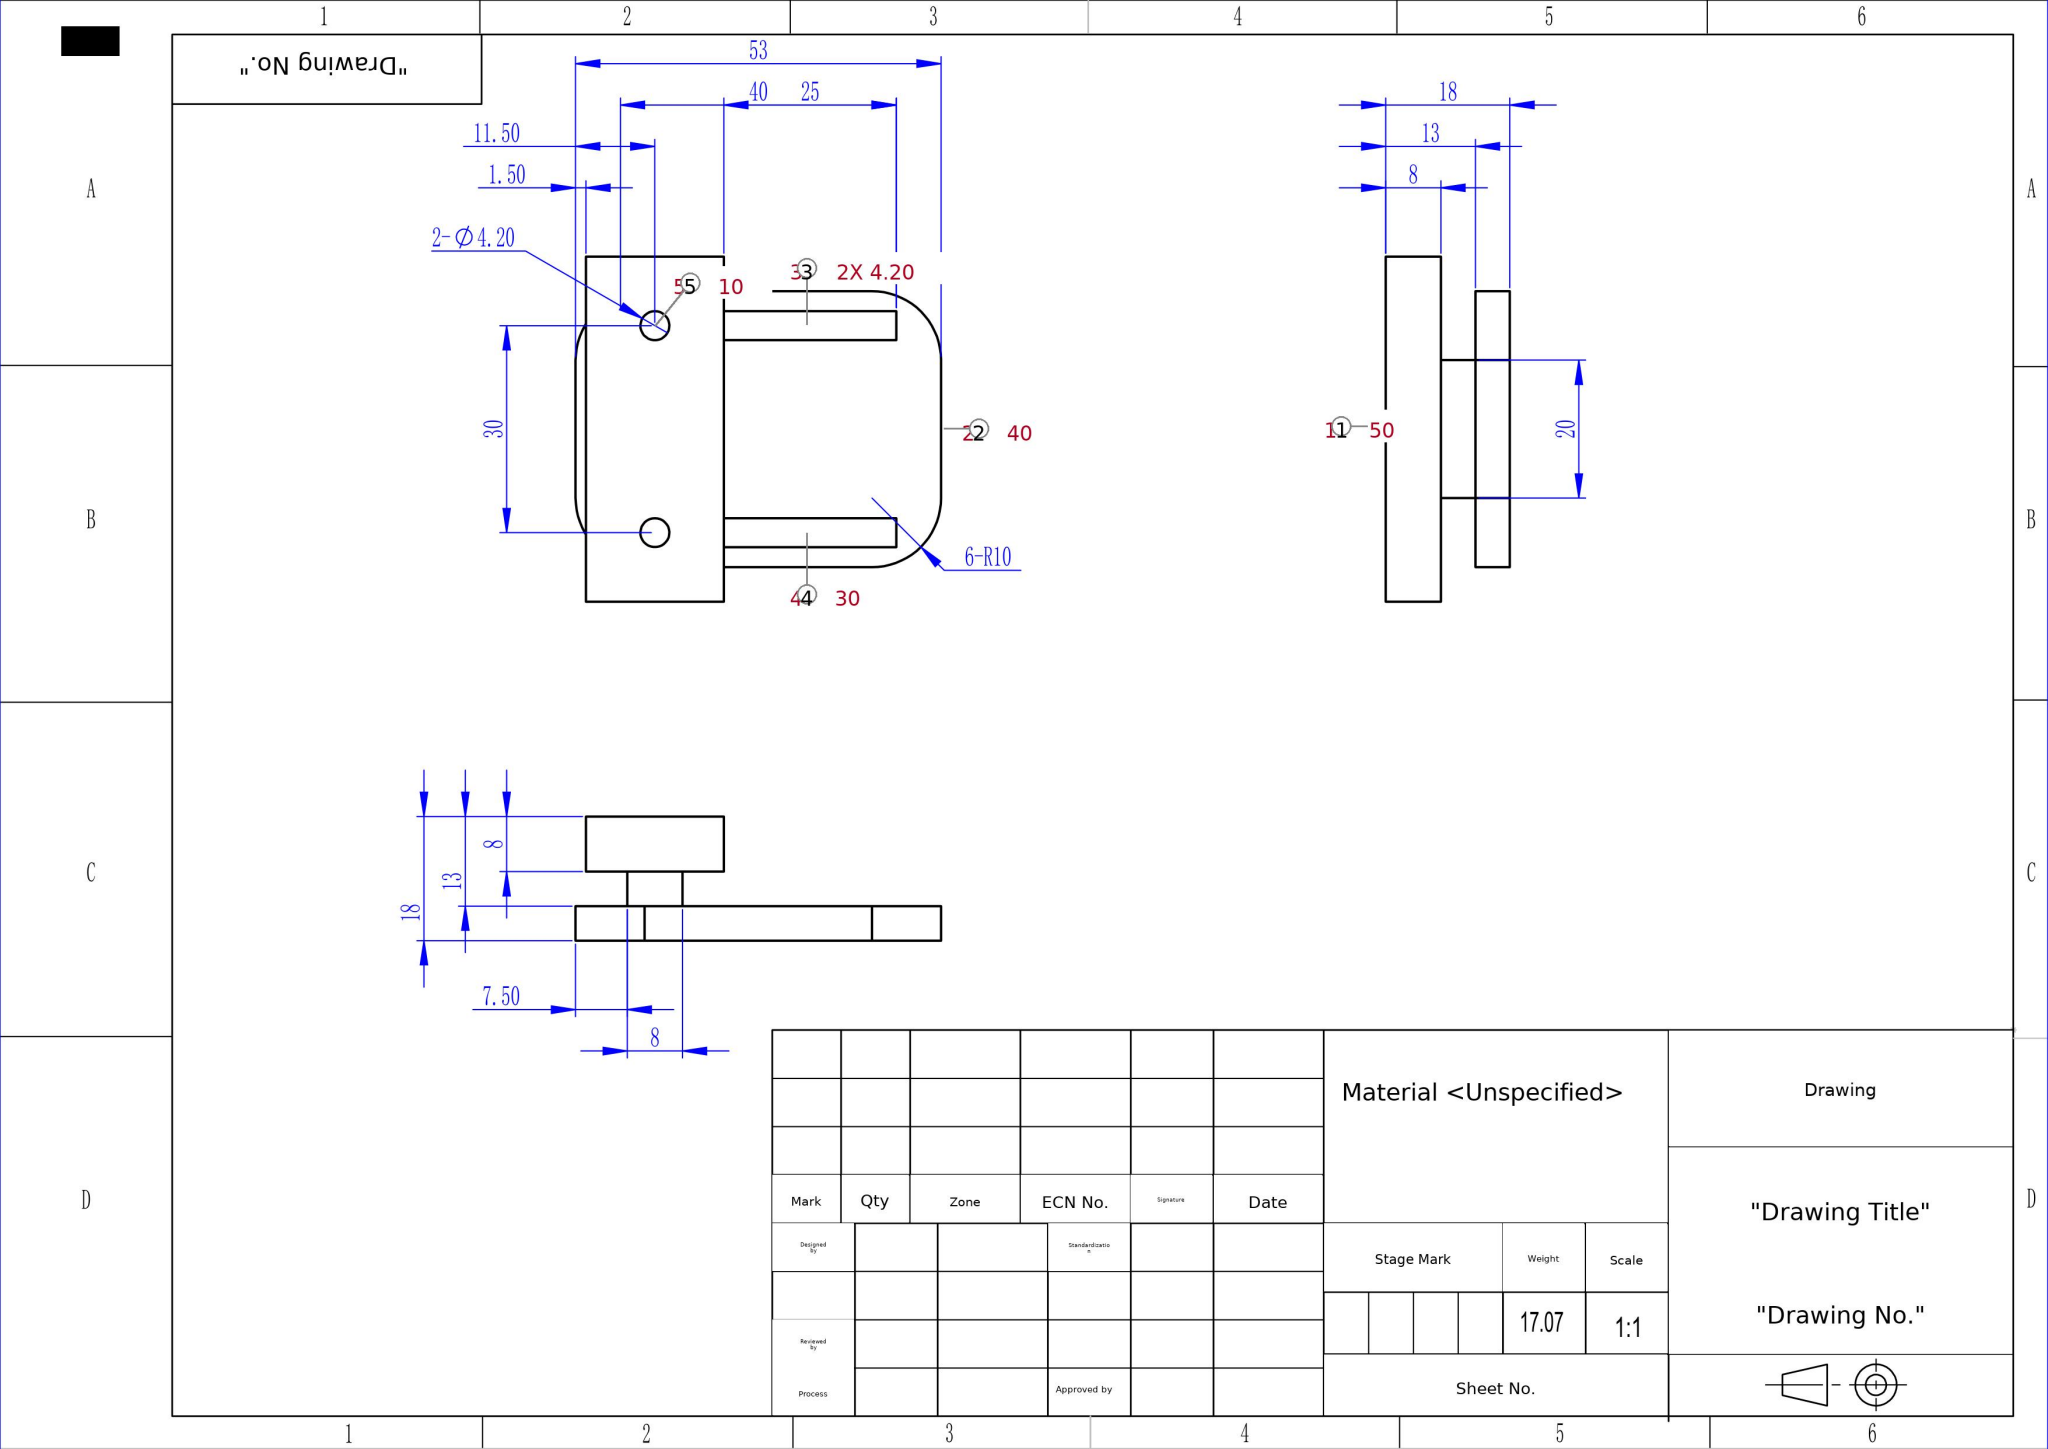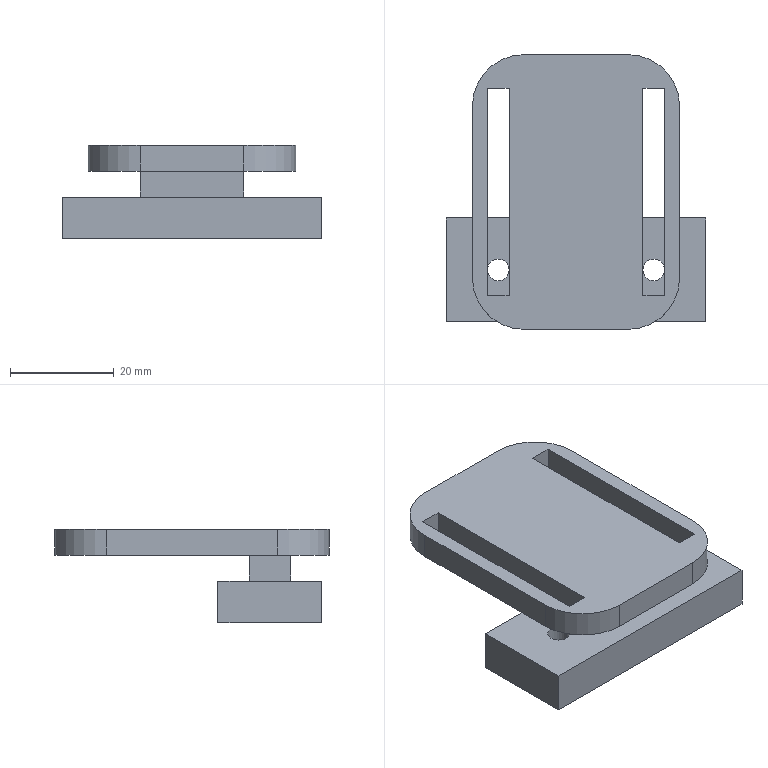Part | SolidWorks | mm | material Unspecified | 1 solid | 32 faces | box 50 x 53 x 18 mm | volume 17069 mm3 | plane 24 | cylinder 8 | commonest cylinder face diameters 4.2 x4 20 x4
build123d program:
from build123d import *

# Parameters (mm, degrees)
SKETCH1_W           = 50
SKETCH1_H           = 20
SKETCH1_R           = 2.1
BOSS_EXTRUDE1_DEPTH = 8
SKETCH2_W           = 20
SKETCH2_H           = 8
BOSS_EXTRUDE2_DEPTH = 5
SKETCH3_W           = 40
SKETCH3_H           = 53
SKETCH3_W_2         = 4.2
SKETCH3_H_2         = 40
BOSS_EXTRUDE3_DEPTH = 5
FILLET1_R           = 10


with BuildPart() as part:
    # Sketch1 → Boss-Extrude1 (new body)
    with BuildSketch(Plane.XY):
        Rectangle(SKETCH1_W, SKETCH1_H)
        with Locations((-15, 0)):
            Circle(SKETCH1_R, mode=Mode.SUBTRACT)
        with Locations((15, 0)):
            Circle(SKETCH1_R, mode=Mode.SUBTRACT)
    extrude(amount=BOSS_EXTRUDE1_DEPTH)

    # Sketch2 → Boss-Extrude2 (add)
    with BuildSketch(Plane.XY.offset(8)):
        Rectangle(SKETCH2_W, SKETCH2_H)
    extrude(amount=BOSS_EXTRUDE2_DEPTH)

    # Sketch3 → Boss-Extrude3 (add)
    with BuildSketch(Plane.XY.offset(13)):
        with Locations((0, 15)):
            Rectangle(SKETCH3_W, SKETCH3_H)
        with Locations((-15, 15)):
            Rectangle(SKETCH3_W_2, SKETCH3_H_2, mode=Mode.SUBTRACT)
        with Locations((15, 15)):
            Rectangle(SKETCH3_W_2, SKETCH3_H_2, mode=Mode.SUBTRACT)
    extrude(amount=BOSS_EXTRUDE3_DEPTH)

    # Fillet1
    fillet1_edges = [part.edges().sort_by_distance(p)[0] for p in [
        (20, -11.5, 15.5),
        (20, 41.5, 15.5),
        (-20, 41.5, 15.5),
        (-20, -11.5, 15.5),
    ]]
    fillet(fillet1_edges, radius=FILLET1_R)


solid = part.part
STEP:
#1=CARTESIAN_POINT('',(12.9,0.,8.));
#2=VERTEX_POINT('',#1);
#3=CARTESIAN_POINT('',(17.1,0.,8.));
#4=VERTEX_POINT('',#3);
#5=CARTESIAN_POINT('',(15.,0.,8.));
#6=DIRECTION('',(0.,0.,1.));
#7=DIRECTION('',(1.,0.,0.));
#8=AXIS2_PLACEMENT_3D('',#5,#6,#7);
#9=CIRCLE('',#8,2.1);
#10=EDGE_CURVE('',#2,#4,#9,.T.);
#11=ORIENTED_EDGE('',*,*,#10,.T.);
#12=CARTESIAN_POINT('',(17.1,0.,0.));
#13=VERTEX_POINT('',#12);
#14=CARTESIAN_POINT('',(17.1,0.,8.));
#15=DIRECTION('',(0.,0.,-1.));
#16=VECTOR('',#15,1000.);
#17=LINE('',#14,#16);
#18=EDGE_CURVE('',#4,#13,#17,.T.);
#19=ORIENTED_EDGE('',*,*,#18,.T.);
#20=CARTESIAN_POINT('',(12.9,0.,0.));
#21=VERTEX_POINT('',#20);
#22=CARTESIAN_POINT('',(15.,0.,0.));
#23=DIRECTION('',(0.,0.,1.));
#24=DIRECTION('',(1.,0.,0.));
#25=AXIS2_PLACEMENT_3D('',#22,#23,#24);
#26=CIRCLE('',#25,2.1);
#27=EDGE_CURVE('',#21,#13,#26,.T.);
#28=ORIENTED_EDGE('',*,*,#27,.F.);
#29=CARTESIAN_POINT('',(12.9,0.,8.));
#30=DIRECTION('',(0.,0.,-1.));
#31=VECTOR('',#30,1000.);
#32=LINE('',#29,#31);
#33=EDGE_CURVE('',#2,#21,#32,.T.);
#34=ORIENTED_EDGE('',*,*,#33,.F.);
#35=EDGE_LOOP('',(#11,#19,#28,#34));
#36=FACE_OUTER_BOUND('',#35,.T.);
#37=CARTESIAN_POINT('',(15.,0.,8.));
#38=DIRECTION('',(0.,0.,-1.));
#39=DIRECTION('',(-1.,0.,0.));
#40=AXIS2_PLACEMENT_3D('',#37,#38,#39);
#41=CYLINDRICAL_SURFACE('',#40,2.1);
#42=ADVANCED_FACE('',(#36),#41,.F.);
#43=CARTESIAN_POINT('',(-17.1,0.,8.));
#44=VERTEX_POINT('',#43);
#45=CARTESIAN_POINT('',(-12.9,0.,8.));
#46=VERTEX_POINT('',#45);
#47=CARTESIAN_POINT('',(-15.,0.,8.));
#48=DIRECTION('',(0.,0.,1.));
#49=DIRECTION('',(1.,0.,0.));
#50=AXIS2_PLACEMENT_3D('',#47,#48,#49);
#51=CIRCLE('',#50,2.1);
#52=EDGE_CURVE('',#44,#46,#51,.T.);
#53=ORIENTED_EDGE('',*,*,#52,.T.);
#54=CARTESIAN_POINT('',(-12.9,0.,0.));
#55=VERTEX_POINT('',#54);
#56=CARTESIAN_POINT('',(-12.9,0.,8.));
#57=DIRECTION('',(0.,0.,-1.));
#58=VECTOR('',#57,1000.);
#59=LINE('',#56,#58);
#60=EDGE_CURVE('',#46,#55,#59,.T.);
#61=ORIENTED_EDGE('',*,*,#60,.T.);
#62=CARTESIAN_POINT('',(-17.1,0.,0.));
#63=VERTEX_POINT('',#62);
#64=CARTESIAN_POINT('',(-15.,0.,0.));
#65=DIRECTION('',(0.,0.,1.));
#66=DIRECTION('',(1.,0.,0.));
#67=AXIS2_PLACEMENT_3D('',#64,#65,#66);
#68=CIRCLE('',#67,2.1);
#69=EDGE_CURVE('',#63,#55,#68,.T.);
#70=ORIENTED_EDGE('',*,*,#69,.F.);
#71=CARTESIAN_POINT('',(-17.1,0.,8.));
#72=DIRECTION('',(0.,0.,-1.));
#73=VECTOR('',#72,1000.);
#74=LINE('',#71,#73);
#75=EDGE_CURVE('',#44,#63,#74,.T.);
#76=ORIENTED_EDGE('',*,*,#75,.F.);
#77=EDGE_LOOP('',(#53,#61,#70,#76));
#78=FACE_OUTER_BOUND('',#77,.T.);
#79=CARTESIAN_POINT('',(-15.,0.,8.));
#80=DIRECTION('',(0.,0.,-1.));
#81=DIRECTION('',(-1.,0.,0.));
#82=AXIS2_PLACEMENT_3D('',#79,#80,#81);
#83=CYLINDRICAL_SURFACE('',#82,2.1);
#84=ADVANCED_FACE('',(#78),#83,.F.);
#85=ORIENTED_EDGE('',*,*,#52,.F.);
#86=CARTESIAN_POINT('',(-15.,0.,8.));
#87=DIRECTION('',(0.,0.,1.));
#88=DIRECTION('',(1.,0.,0.));
#89=AXIS2_PLACEMENT_3D('',#86,#87,#88);
#90=CIRCLE('',#89,2.1);
#91=EDGE_CURVE('',#46,#44,#90,.T.);
#92=ORIENTED_EDGE('',*,*,#91,.F.);
#93=EDGE_LOOP('',(#85,#92));
#94=FACE_BOUND('',#93,.T.);
#95=CARTESIAN_POINT('',(25.,-10.,8.));
#96=VERTEX_POINT('',#95);
#97=CARTESIAN_POINT('',(25.,10.,8.));
#98=VERTEX_POINT('',#97);
#99=CARTESIAN_POINT('',(25.,10.,8.));
#100=DIRECTION('',(-0.,1.,0.));
#101=VECTOR('',#100,1000.);
#102=LINE('',#99,#101);
#103=EDGE_CURVE('',#96,#98,#102,.T.);
#104=ORIENTED_EDGE('',*,*,#103,.T.);
#105=CARTESIAN_POINT('',(-25.,10.,8.));
#106=VERTEX_POINT('',#105);
#107=CARTESIAN_POINT('',(-25.,10.,8.));
#108=DIRECTION('',(-1.,0.,0.));
#109=VECTOR('',#108,1000.);
#110=LINE('',#107,#109);
#111=EDGE_CURVE('',#98,#106,#110,.T.);
#112=ORIENTED_EDGE('',*,*,#111,.T.);
#113=CARTESIAN_POINT('',(-25.,-10.,8.));
#114=VERTEX_POINT('',#113);
#115=CARTESIAN_POINT('',(-25.,10.,8.));
#116=DIRECTION('',(0.,-1.,0.));
#117=VECTOR('',#116,1000.);
#118=LINE('',#115,#117);
#119=EDGE_CURVE('',#106,#114,#118,.T.);
#120=ORIENTED_EDGE('',*,*,#119,.T.);
#121=CARTESIAN_POINT('',(-25.,-10.,8.));
#122=DIRECTION('',(1.,0.,0.));
#123=VECTOR('',#122,1000.);
#124=LINE('',#121,#123);
#125=EDGE_CURVE('',#114,#96,#124,.T.);
#126=ORIENTED_EDGE('',*,*,#125,.T.);
#127=EDGE_LOOP('',(#104,#112,#120,#126));
#128=FACE_OUTER_BOUND('',#127,.T.);
#129=ORIENTED_EDGE('',*,*,#10,.F.);
#130=CARTESIAN_POINT('',(15.,0.,8.));
#131=DIRECTION('',(0.,0.,1.));
#132=DIRECTION('',(1.,0.,0.));
#133=AXIS2_PLACEMENT_3D('',#130,#131,#132);
#134=CIRCLE('',#133,2.1);
#135=EDGE_CURVE('',#4,#2,#134,.T.);
#136=ORIENTED_EDGE('',*,*,#135,.F.);
#137=EDGE_LOOP('',(#129,#136));
#138=FACE_BOUND('',#137,.T.);
#139=CARTESIAN_POINT('',(10.,4.,8.));
#140=VERTEX_POINT('',#139);
#141=CARTESIAN_POINT('',(-10.,4.,8.));
#142=VERTEX_POINT('',#141);
#143=CARTESIAN_POINT('',(-10.,4.,8.));
#144=DIRECTION('',(-1.,0.,0.));
#145=VECTOR('',#144,1000.);
#146=LINE('',#143,#145);
#147=EDGE_CURVE('',#140,#142,#146,.T.);
#148=ORIENTED_EDGE('',*,*,#147,.F.);
#149=CARTESIAN_POINT('',(10.,-4.,8.));
#150=VERTEX_POINT('',#149);
#151=CARTESIAN_POINT('',(10.,4.,8.));
#152=DIRECTION('',(-0.,1.,0.));
#153=VECTOR('',#152,1000.);
#154=LINE('',#151,#153);
#155=EDGE_CURVE('',#150,#140,#154,.T.);
#156=ORIENTED_EDGE('',*,*,#155,.F.);
#157=CARTESIAN_POINT('',(-10.,-4.,8.));
#158=VERTEX_POINT('',#157);
#159=CARTESIAN_POINT('',(-10.,-4.,8.));
#160=DIRECTION('',(1.,0.,0.));
#161=VECTOR('',#160,1000.);
#162=LINE('',#159,#161);
#163=EDGE_CURVE('',#158,#150,#162,.T.);
#164=ORIENTED_EDGE('',*,*,#163,.F.);
#165=CARTESIAN_POINT('',(-10.,4.,8.));
#166=DIRECTION('',(0.,-1.,0.));
#167=VECTOR('',#166,1000.);
#168=LINE('',#165,#167);
#169=EDGE_CURVE('',#142,#158,#168,.T.);
#170=ORIENTED_EDGE('',*,*,#169,.F.);
#171=EDGE_LOOP('',(#148,#156,#164,#170));
#172=FACE_BOUND('',#171,.T.);
#173=CARTESIAN_POINT('',(0.,0.,8.));
#174=DIRECTION('',(0.,0.,1.));
#175=DIRECTION('',(1.,0.,0.));
#176=AXIS2_PLACEMENT_3D('',#173,#174,#175);
#177=PLANE('',#176);
#178=ADVANCED_FACE('',(#94,#128,#138,#172),#177,.T.);
#179=CARTESIAN_POINT('',(25.,-10.,0.));
#180=VERTEX_POINT('',#179);
#181=CARTESIAN_POINT('',(25.,10.,0.));
#182=VERTEX_POINT('',#181);
#183=CARTESIAN_POINT('',(25.,10.,0.));
#184=DIRECTION('',(-0.,1.,0.));
#185=VECTOR('',#184,1000.);
#186=LINE('',#183,#185);
#187=EDGE_CURVE('',#180,#182,#186,.T.);
#188=ORIENTED_EDGE('',*,*,#187,.F.);
#189=CARTESIAN_POINT('',(-25.,-10.,0.));
#190=VERTEX_POINT('',#189);
#191=CARTESIAN_POINT('',(-25.,-10.,0.));
#192=DIRECTION('',(1.,0.,0.));
#193=VECTOR('',#192,1000.);
#194=LINE('',#191,#193);
#195=EDGE_CURVE('',#190,#180,#194,.T.);
#196=ORIENTED_EDGE('',*,*,#195,.F.);
#197=CARTESIAN_POINT('',(-25.,10.,0.));
#198=VERTEX_POINT('',#197);
#199=CARTESIAN_POINT('',(-25.,10.,0.));
#200=DIRECTION('',(0.,-1.,0.));
#201=VECTOR('',#200,1000.);
#202=LINE('',#199,#201);
#203=EDGE_CURVE('',#198,#190,#202,.T.);
#204=ORIENTED_EDGE('',*,*,#203,.F.);
#205=CARTESIAN_POINT('',(-25.,10.,0.));
#206=DIRECTION('',(-1.,0.,0.));
#207=VECTOR('',#206,1000.);
#208=LINE('',#205,#207);
#209=EDGE_CURVE('',#182,#198,#208,.T.);
#210=ORIENTED_EDGE('',*,*,#209,.F.);
#211=EDGE_LOOP('',(#188,#196,#204,#210));
#212=FACE_OUTER_BOUND('',#211,.T.);
#213=ORIENTED_EDGE('',*,*,#69,.T.);
#214=CARTESIAN_POINT('',(-15.,0.,0.));
#215=DIRECTION('',(0.,0.,1.));
#216=DIRECTION('',(1.,0.,0.));
#217=AXIS2_PLACEMENT_3D('',#214,#215,#216);
#218=CIRCLE('',#217,2.1);
#219=EDGE_CURVE('',#55,#63,#218,.T.);
#220=ORIENTED_EDGE('',*,*,#219,.T.);
#221=EDGE_LOOP('',(#213,#220));
#222=FACE_BOUND('',#221,.T.);
#223=ORIENTED_EDGE('',*,*,#27,.T.);
#224=CARTESIAN_POINT('',(15.,0.,0.));
#225=DIRECTION('',(0.,0.,1.));
#226=DIRECTION('',(1.,0.,0.));
#227=AXIS2_PLACEMENT_3D('',#224,#225,#226);
#228=CIRCLE('',#227,2.1);
#229=EDGE_CURVE('',#13,#21,#228,.T.);
#230=ORIENTED_EDGE('',*,*,#229,.T.);
#231=EDGE_LOOP('',(#223,#230));
#232=FACE_BOUND('',#231,.T.);
#233=CARTESIAN_POINT('',(0.,0.,0.));
#234=DIRECTION('',(0.,0.,1.));
#235=DIRECTION('',(1.,0.,0.));
#236=AXIS2_PLACEMENT_3D('',#233,#234,#235);
#237=PLANE('',#236);
#238=ADVANCED_FACE('',(#212,#222,#232),#237,.F.);
#239=ORIENTED_EDGE('',*,*,#187,.T.);
#240=CARTESIAN_POINT('',(25.,10.,8.));
#241=DIRECTION('',(0.,0.,-1.));
#242=VECTOR('',#241,1000.);
#243=LINE('',#240,#242);
#244=EDGE_CURVE('',#98,#182,#243,.T.);
#245=ORIENTED_EDGE('',*,*,#244,.F.);
#246=ORIENTED_EDGE('',*,*,#103,.F.);
#247=CARTESIAN_POINT('',(25.,-10.,8.));
#248=DIRECTION('',(0.,0.,-1.));
#249=VECTOR('',#248,1000.);
#250=LINE('',#247,#249);
#251=EDGE_CURVE('',#96,#180,#250,.T.);
#252=ORIENTED_EDGE('',*,*,#251,.T.);
#253=EDGE_LOOP('',(#239,#245,#246,#252));
#254=FACE_OUTER_BOUND('',#253,.T.);
#255=CARTESIAN_POINT('',(25.,10.,8.));
#256=DIRECTION('',(-1.,-0.,0.));
#257=DIRECTION('',(0.,-1.,0.));
#258=AXIS2_PLACEMENT_3D('',#255,#256,#257);
#259=PLANE('',#258);
#260=ADVANCED_FACE('',(#254),#259,.F.);
#261=ORIENTED_EDGE('',*,*,#209,.T.);
#262=CARTESIAN_POINT('',(-25.,10.,8.));
#263=DIRECTION('',(0.,0.,-1.));
#264=VECTOR('',#263,1000.);
#265=LINE('',#262,#264);
#266=EDGE_CURVE('',#106,#198,#265,.T.);
#267=ORIENTED_EDGE('',*,*,#266,.F.);
#268=ORIENTED_EDGE('',*,*,#111,.F.);
#269=ORIENTED_EDGE('',*,*,#244,.T.);
#270=EDGE_LOOP('',(#261,#267,#268,#269));
#271=FACE_OUTER_BOUND('',#270,.T.);
#272=CARTESIAN_POINT('',(-25.,10.,8.));
#273=DIRECTION('',(0.,-1.,0.));
#274=DIRECTION('',(0.,0.,-1.));
#275=AXIS2_PLACEMENT_3D('',#272,#273,#274);
#276=PLANE('',#275);
#277=ADVANCED_FACE('',(#271),#276,.F.);
#278=ORIENTED_EDGE('',*,*,#203,.T.);
#279=CARTESIAN_POINT('',(-25.,-10.,8.));
#280=DIRECTION('',(0.,0.,-1.));
#281=VECTOR('',#280,1000.);
#282=LINE('',#279,#281);
#283=EDGE_CURVE('',#114,#190,#282,.T.);
#284=ORIENTED_EDGE('',*,*,#283,.F.);
#285=ORIENTED_EDGE('',*,*,#119,.F.);
#286=ORIENTED_EDGE('',*,*,#266,.T.);
#287=EDGE_LOOP('',(#278,#284,#285,#286));
#288=FACE_OUTER_BOUND('',#287,.T.);
#289=CARTESIAN_POINT('',(-25.,10.,8.));
#290=DIRECTION('',(1.,0.,0.));
#291=DIRECTION('',(0.,0.,-1.));
#292=AXIS2_PLACEMENT_3D('',#289,#290,#291);
#293=PLANE('',#292);
#294=ADVANCED_FACE('',(#288),#293,.F.);
#295=ORIENTED_EDGE('',*,*,#195,.T.);
#296=ORIENTED_EDGE('',*,*,#251,.F.);
#297=ORIENTED_EDGE('',*,*,#125,.F.);
#298=ORIENTED_EDGE('',*,*,#283,.T.);
#299=EDGE_LOOP('',(#295,#296,#297,#298));
#300=FACE_OUTER_BOUND('',#299,.T.);
#301=CARTESIAN_POINT('',(-25.,-10.,8.));
#302=DIRECTION('',(0.,1.,0.));
#303=DIRECTION('',(0.,0.,1.));
#304=AXIS2_PLACEMENT_3D('',#301,#302,#303);
#305=PLANE('',#304);
#306=ADVANCED_FACE('',(#300),#305,.F.);
#307=ORIENTED_EDGE('',*,*,#60,.F.);
#308=ORIENTED_EDGE('',*,*,#91,.T.);
#309=ORIENTED_EDGE('',*,*,#75,.T.);
#310=ORIENTED_EDGE('',*,*,#219,.F.);
#311=EDGE_LOOP('',(#307,#308,#309,#310));
#312=FACE_OUTER_BOUND('',#311,.T.);
#313=CARTESIAN_POINT('',(-15.,0.,8.));
#314=DIRECTION('',(0.,0.,-1.));
#315=DIRECTION('',(-1.,0.,0.));
#316=AXIS2_PLACEMENT_3D('',#313,#314,#315);
#317=CYLINDRICAL_SURFACE('',#316,2.1);
#318=ADVANCED_FACE('',(#312),#317,.F.);
#319=ORIENTED_EDGE('',*,*,#18,.F.);
#320=ORIENTED_EDGE('',*,*,#135,.T.);
#321=ORIENTED_EDGE('',*,*,#33,.T.);
#322=ORIENTED_EDGE('',*,*,#229,.F.);
#323=EDGE_LOOP('',(#319,#320,#321,#322));
#324=FACE_OUTER_BOUND('',#323,.T.);
#325=CARTESIAN_POINT('',(15.,0.,8.));
#326=DIRECTION('',(0.,0.,-1.));
#327=DIRECTION('',(-1.,0.,0.));
#328=AXIS2_PLACEMENT_3D('',#325,#326,#327);
#329=CYLINDRICAL_SURFACE('',#328,2.1);
#330=ADVANCED_FACE('',(#324),#329,.F.);
#331=ORIENTED_EDGE('',*,*,#155,.T.);
#332=CARTESIAN_POINT('',(10.,4.,13.));
#333=VERTEX_POINT('',#332);
#334=CARTESIAN_POINT('',(10.,4.,13.));
#335=DIRECTION('',(0.,0.,-1.));
#336=VECTOR('',#335,1000.);
#337=LINE('',#334,#336);
#338=EDGE_CURVE('',#333,#140,#337,.T.);
#339=ORIENTED_EDGE('',*,*,#338,.F.);
#340=CARTESIAN_POINT('',(10.,-4.,13.));
#341=VERTEX_POINT('',#340);
#342=CARTESIAN_POINT('',(10.,4.,13.));
#343=DIRECTION('',(-0.,1.,0.));
#344=VECTOR('',#343,1000.);
#345=LINE('',#342,#344);
#346=EDGE_CURVE('',#341,#333,#345,.T.);
#347=ORIENTED_EDGE('',*,*,#346,.F.);
#348=CARTESIAN_POINT('',(10.,-4.,13.));
#349=DIRECTION('',(0.,0.,-1.));
#350=VECTOR('',#349,1000.);
#351=LINE('',#348,#350);
#352=EDGE_CURVE('',#341,#150,#351,.T.);
#353=ORIENTED_EDGE('',*,*,#352,.T.);
#354=EDGE_LOOP('',(#331,#339,#347,#353));
#355=FACE_OUTER_BOUND('',#354,.T.);
#356=CARTESIAN_POINT('',(10.,4.,13.));
#357=DIRECTION('',(-1.,-0.,0.));
#358=DIRECTION('',(0.,-1.,0.));
#359=AXIS2_PLACEMENT_3D('',#356,#357,#358);
#360=PLANE('',#359);
#361=ADVANCED_FACE('',(#355),#360,.F.);
#362=ORIENTED_EDGE('',*,*,#147,.T.);
#363=CARTESIAN_POINT('',(-10.,4.,13.));
#364=VERTEX_POINT('',#363);
#365=CARTESIAN_POINT('',(-10.,4.,13.));
#366=DIRECTION('',(0.,0.,-1.));
#367=VECTOR('',#366,1000.);
#368=LINE('',#365,#367);
#369=EDGE_CURVE('',#364,#142,#368,.T.);
#370=ORIENTED_EDGE('',*,*,#369,.F.);
#371=CARTESIAN_POINT('',(-10.,4.,13.));
#372=DIRECTION('',(-1.,0.,0.));
#373=VECTOR('',#372,1000.);
#374=LINE('',#371,#373);
#375=EDGE_CURVE('',#333,#364,#374,.T.);
#376=ORIENTED_EDGE('',*,*,#375,.F.);
#377=ORIENTED_EDGE('',*,*,#338,.T.);
#378=EDGE_LOOP('',(#362,#370,#376,#377));
#379=FACE_OUTER_BOUND('',#378,.T.);
#380=CARTESIAN_POINT('',(-10.,4.,13.));
#381=DIRECTION('',(0.,-1.,0.));
#382=DIRECTION('',(0.,0.,-1.));
#383=AXIS2_PLACEMENT_3D('',#380,#381,#382);
#384=PLANE('',#383);
#385=ADVANCED_FACE('',(#379),#384,.F.);
#386=ORIENTED_EDGE('',*,*,#169,.T.);
#387=CARTESIAN_POINT('',(-10.,-4.,13.));
#388=VERTEX_POINT('',#387);
#389=CARTESIAN_POINT('',(-10.,-4.,13.));
#390=DIRECTION('',(0.,0.,-1.));
#391=VECTOR('',#390,1000.);
#392=LINE('',#389,#391);
#393=EDGE_CURVE('',#388,#158,#392,.T.);
#394=ORIENTED_EDGE('',*,*,#393,.F.);
#395=CARTESIAN_POINT('',(-10.,4.,13.));
#396=DIRECTION('',(0.,-1.,0.));
#397=VECTOR('',#396,1000.);
#398=LINE('',#395,#397);
#399=EDGE_CURVE('',#364,#388,#398,.T.);
#400=ORIENTED_EDGE('',*,*,#399,.F.);
#401=ORIENTED_EDGE('',*,*,#369,.T.);
#402=EDGE_LOOP('',(#386,#394,#400,#401));
#403=FACE_OUTER_BOUND('',#402,.T.);
#404=CARTESIAN_POINT('',(-10.,4.,13.));
#405=DIRECTION('',(1.,0.,0.));
#406=DIRECTION('',(-0.,1.,0.));
#407=AXIS2_PLACEMENT_3D('',#404,#405,#406);
#408=PLANE('',#407);
#409=ADVANCED_FACE('',(#403),#408,.F.);
#410=ORIENTED_EDGE('',*,*,#163,.T.);
#411=ORIENTED_EDGE('',*,*,#352,.F.);
#412=CARTESIAN_POINT('',(-10.,-4.,13.));
#413=DIRECTION('',(1.,0.,0.));
#414=VECTOR('',#413,1000.);
#415=LINE('',#412,#414);
#416=EDGE_CURVE('',#388,#341,#415,.T.);
#417=ORIENTED_EDGE('',*,*,#416,.F.);
#418=ORIENTED_EDGE('',*,*,#393,.T.);
#419=EDGE_LOOP('',(#410,#411,#417,#418));
#420=FACE_OUTER_BOUND('',#419,.T.);
#421=CARTESIAN_POINT('',(-10.,-4.,13.));
#422=DIRECTION('',(0.,1.,0.));
#423=DIRECTION('',(0.,0.,1.));
#424=AXIS2_PLACEMENT_3D('',#421,#422,#423);
#425=PLANE('',#424);
#426=ADVANCED_FACE('',(#420),#425,.F.);
#427=CARTESIAN_POINT('',(-17.1,35.,13.));
#428=VERTEX_POINT('',#427);
#429=CARTESIAN_POINT('',(-17.1,-5.,13.));
#430=VERTEX_POINT('',#429);
#431=CARTESIAN_POINT('',(-17.1,35.,13.));
#432=DIRECTION('',(0.,-1.,0.));
#433=VECTOR('',#432,1000.);
#434=LINE('',#431,#433);
#435=EDGE_CURVE('',#428,#430,#434,.T.);
#436=ORIENTED_EDGE('',*,*,#435,.T.);
#437=CARTESIAN_POINT('',(-12.9,-5.,13.));
#438=VERTEX_POINT('',#437);
#439=CARTESIAN_POINT('',(-17.1,-5.,13.));
#440=DIRECTION('',(1.,0.,0.));
#441=VECTOR('',#440,1000.);
#442=LINE('',#439,#441);
#443=EDGE_CURVE('',#430,#438,#442,.T.);
#444=ORIENTED_EDGE('',*,*,#443,.T.);
#445=CARTESIAN_POINT('',(-12.9,35.,13.));
#446=VERTEX_POINT('',#445);
#447=CARTESIAN_POINT('',(-12.9,35.,13.));
#448=DIRECTION('',(-0.,1.,0.));
#449=VECTOR('',#448,1000.);
#450=LINE('',#447,#449);
#451=EDGE_CURVE('',#438,#446,#450,.T.);
#452=ORIENTED_EDGE('',*,*,#451,.T.);
#453=CARTESIAN_POINT('',(-17.1,35.,13.));
#454=DIRECTION('',(-1.,0.,0.));
#455=VECTOR('',#454,1000.);
#456=LINE('',#453,#455);
#457=EDGE_CURVE('',#446,#428,#456,.T.);
#458=ORIENTED_EDGE('',*,*,#457,.T.);
#459=EDGE_LOOP('',(#436,#444,#452,#458));
#460=FACE_BOUND('',#459,.T.);
#461=CARTESIAN_POINT('',(20.,-1.5,13.));
#462=VERTEX_POINT('',#461);
#463=CARTESIAN_POINT('',(20.,31.5,13.));
#464=VERTEX_POINT('',#463);
#465=CARTESIAN_POINT('',(20.,41.5,13.));
#466=DIRECTION('',(-0.,1.,0.));
#467=VECTOR('',#466,1000.);
#468=LINE('',#465,#467);
#469=EDGE_CURVE('',#462,#464,#468,.T.);
#470=ORIENTED_EDGE('',*,*,#469,.F.);
#471=CARTESIAN_POINT('',(10.,-11.5,13.));
#472=VERTEX_POINT('',#471);
#473=CARTESIAN_POINT('',(10.,-1.5,13.));
#474=DIRECTION('',(0.,0.,-1.));
#475=DIRECTION('',(1.,0.,0.));
#476=AXIS2_PLACEMENT_3D('',#473,#474,#475);
#477=CIRCLE('',#476,10.);
#478=EDGE_CURVE('',#462,#472,#477,.T.);
#479=ORIENTED_EDGE('',*,*,#478,.T.);
#480=CARTESIAN_POINT('',(-10.,-11.5,13.));
#481=VERTEX_POINT('',#480);
#482=CARTESIAN_POINT('',(-20.,-11.5,13.));
#483=DIRECTION('',(1.,0.,0.));
#484=VECTOR('',#483,1000.);
#485=LINE('',#482,#484);
#486=EDGE_CURVE('',#481,#472,#485,.T.);
#487=ORIENTED_EDGE('',*,*,#486,.F.);
#488=CARTESIAN_POINT('',(-20.,-1.5,13.));
#489=VERTEX_POINT('',#488);
#490=CARTESIAN_POINT('',(-10.,-1.5,13.));
#491=DIRECTION('',(0.,0.,-1.));
#492=DIRECTION('',(1.,0.,0.));
#493=AXIS2_PLACEMENT_3D('',#490,#491,#492);
#494=CIRCLE('',#493,10.);
#495=EDGE_CURVE('',#481,#489,#494,.T.);
#496=ORIENTED_EDGE('',*,*,#495,.T.);
#497=CARTESIAN_POINT('',(-20.,31.5,13.));
#498=VERTEX_POINT('',#497);
#499=CARTESIAN_POINT('',(-20.,41.5,13.));
#500=DIRECTION('',(0.,-1.,0.));
#501=VECTOR('',#500,1000.);
#502=LINE('',#499,#501);
#503=EDGE_CURVE('',#498,#489,#502,.T.);
#504=ORIENTED_EDGE('',*,*,#503,.F.);
#505=CARTESIAN_POINT('',(-10.,41.5,13.));
#506=VERTEX_POINT('',#505);
#507=CARTESIAN_POINT('',(-10.,31.5,13.));
#508=DIRECTION('',(0.,0.,-1.));
#509=DIRECTION('',(1.,0.,0.));
#510=AXIS2_PLACEMENT_3D('',#507,#508,#509);
#511=CIRCLE('',#510,10.);
#512=EDGE_CURVE('',#498,#506,#511,.T.);
#513=ORIENTED_EDGE('',*,*,#512,.T.);
#514=CARTESIAN_POINT('',(10.,41.5,13.));
#515=VERTEX_POINT('',#514);
#516=CARTESIAN_POINT('',(-20.,41.5,13.));
#517=DIRECTION('',(-1.,0.,0.));
#518=VECTOR('',#517,1000.);
#519=LINE('',#516,#518);
#520=EDGE_CURVE('',#515,#506,#519,.T.);
#521=ORIENTED_EDGE('',*,*,#520,.F.);
#522=CARTESIAN_POINT('',(10.,31.5,13.));
#523=DIRECTION('',(0.,0.,-1.));
#524=DIRECTION('',(1.,-0.,0.));
#525=AXIS2_PLACEMENT_3D('',#522,#523,#524);
#526=CIRCLE('',#525,10.);
#527=EDGE_CURVE('',#515,#464,#526,.T.);
#528=ORIENTED_EDGE('',*,*,#527,.T.);
#529=EDGE_LOOP('',(#470,#479,#487,#496,#504,#513,#521,#528));
#530=FACE_OUTER_BOUND('',#529,.T.);
#531=CARTESIAN_POINT('',(17.1,35.,13.));
#532=VERTEX_POINT('',#531);
#533=CARTESIAN_POINT('',(12.9,35.,13.));
#534=VERTEX_POINT('',#533);
#535=CARTESIAN_POINT('',(17.1,35.,13.));
#536=DIRECTION('',(-1.,0.,0.));
#537=VECTOR('',#536,1000.);
#538=LINE('',#535,#537);
#539=EDGE_CURVE('',#532,#534,#538,.T.);
#540=ORIENTED_EDGE('',*,*,#539,.T.);
#541=CARTESIAN_POINT('',(12.9,-5.,13.));
#542=VERTEX_POINT('',#541);
#543=CARTESIAN_POINT('',(12.9,35.,13.));
#544=DIRECTION('',(-0.,-1.,0.));
#545=VECTOR('',#544,1000.);
#546=LINE('',#543,#545);
#547=EDGE_CURVE('',#534,#542,#546,.T.);
#548=ORIENTED_EDGE('',*,*,#547,.T.);
#549=CARTESIAN_POINT('',(17.1,-5.,13.));
#550=VERTEX_POINT('',#549);
#551=CARTESIAN_POINT('',(17.1,-5.,13.));
#552=DIRECTION('',(1.,0.,0.));
#553=VECTOR('',#552,1000.);
#554=LINE('',#551,#553);
#555=EDGE_CURVE('',#542,#550,#554,.T.);
#556=ORIENTED_EDGE('',*,*,#555,.T.);
#557=CARTESIAN_POINT('',(17.1,35.,13.));
#558=DIRECTION('',(0.,1.,0.));
#559=VECTOR('',#558,1000.);
#560=LINE('',#557,#559);
#561=EDGE_CURVE('',#550,#532,#560,.T.);
#562=ORIENTED_EDGE('',*,*,#561,.T.);
#563=EDGE_LOOP('',(#540,#548,#556,#562));
#564=FACE_BOUND('',#563,.T.);
#565=ORIENTED_EDGE('',*,*,#416,.T.);
#566=ORIENTED_EDGE('',*,*,#346,.T.);
#567=ORIENTED_EDGE('',*,*,#375,.T.);
#568=ORIENTED_EDGE('',*,*,#399,.T.);
#569=EDGE_LOOP('',(#565,#566,#567,#568));
#570=FACE_BOUND('',#569,.T.);
#571=CARTESIAN_POINT('',(0.,0.,13.));
#572=DIRECTION('',(0.,0.,1.));
#573=DIRECTION('',(1.,0.,0.));
#574=AXIS2_PLACEMENT_3D('',#571,#572,#573);
#575=PLANE('',#574);
#576=ADVANCED_FACE('',(#460,#530,#564,#570),#575,.F.);
#577=CARTESIAN_POINT('',(-10.,-11.5,18.));
#578=VERTEX_POINT('',#577);
#579=CARTESIAN_POINT('',(10.,-11.5,18.));
#580=VERTEX_POINT('',#579);
#581=CARTESIAN_POINT('',(-20.,-11.5,18.));
#582=DIRECTION('',(1.,0.,0.));
#583=VECTOR('',#582,1000.);
#584=LINE('',#581,#583);
#585=EDGE_CURVE('',#578,#580,#584,.T.);
#586=ORIENTED_EDGE('',*,*,#585,.T.);
#587=CARTESIAN_POINT('',(20.,-1.5,18.));
#588=VERTEX_POINT('',#587);
#589=CARTESIAN_POINT('',(10.,-1.5,18.));
#590=DIRECTION('',(0.,0.,1.));
#591=DIRECTION('',(1.,0.,0.));
#592=AXIS2_PLACEMENT_3D('',#589,#590,#591);
#593=CIRCLE('',#592,10.);
#594=EDGE_CURVE('',#580,#588,#593,.T.);
#595=ORIENTED_EDGE('',*,*,#594,.T.);
#596=CARTESIAN_POINT('',(20.,31.5,18.));
#597=VERTEX_POINT('',#596);
#598=CARTESIAN_POINT('',(20.,41.5,18.));
#599=DIRECTION('',(-0.,1.,0.));
#600=VECTOR('',#599,1000.);
#601=LINE('',#598,#600);
#602=EDGE_CURVE('',#588,#597,#601,.T.);
#603=ORIENTED_EDGE('',*,*,#602,.T.);
#604=CARTESIAN_POINT('',(10.,41.5,18.));
#605=VERTEX_POINT('',#604);
#606=CARTESIAN_POINT('',(10.,31.5,18.));
#607=DIRECTION('',(0.,0.,1.));
#608=DIRECTION('',(1.,0.,0.));
#609=AXIS2_PLACEMENT_3D('',#606,#607,#608);
#610=CIRCLE('',#609,10.);
#611=EDGE_CURVE('',#597,#605,#610,.T.);
#612=ORIENTED_EDGE('',*,*,#611,.T.);
#613=CARTESIAN_POINT('',(-10.,41.5,18.));
#614=VERTEX_POINT('',#613);
#615=CARTESIAN_POINT('',(-20.,41.5,18.));
#616=DIRECTION('',(-1.,0.,0.));
#617=VECTOR('',#616,1000.);
#618=LINE('',#615,#617);
#619=EDGE_CURVE('',#605,#614,#618,.T.);
#620=ORIENTED_EDGE('',*,*,#619,.T.);
#621=CARTESIAN_POINT('',(-20.,31.5,18.));
#622=VERTEX_POINT('',#621);
#623=CARTESIAN_POINT('',(-10.,31.5,18.));
#624=DIRECTION('',(0.,0.,1.));
#625=DIRECTION('',(1.,0.,0.));
#626=AXIS2_PLACEMENT_3D('',#623,#624,#625);
#627=CIRCLE('',#626,10.);
#628=EDGE_CURVE('',#614,#622,#627,.T.);
#629=ORIENTED_EDGE('',*,*,#628,.T.);
#630=CARTESIAN_POINT('',(-20.,-1.5,18.));
#631=VERTEX_POINT('',#630);
#632=CARTESIAN_POINT('',(-20.,41.5,18.));
#633=DIRECTION('',(0.,-1.,0.));
#634=VECTOR('',#633,1000.);
#635=LINE('',#632,#634);
#636=EDGE_CURVE('',#622,#631,#635,.T.);
#637=ORIENTED_EDGE('',*,*,#636,.T.);
#638=CARTESIAN_POINT('',(-10.,-1.5,18.));
#639=DIRECTION('',(0.,0.,1.));
#640=DIRECTION('',(1.,0.,0.));
#641=AXIS2_PLACEMENT_3D('',#638,#639,#640);
#642=CIRCLE('',#641,10.);
#643=EDGE_CURVE('',#631,#578,#642,.T.);
#644=ORIENTED_EDGE('',*,*,#643,.T.);
#645=EDGE_LOOP('',(#586,#595,#603,#612,#620,#629,#637,#644));
#646=FACE_OUTER_BOUND('',#645,.T.);
#647=CARTESIAN_POINT('',(-17.1,-5.,18.));
#648=VERTEX_POINT('',#647);
#649=CARTESIAN_POINT('',(-12.9,-5.,18.));
#650=VERTEX_POINT('',#649);
#651=CARTESIAN_POINT('',(-17.1,-5.,18.));
#652=DIRECTION('',(1.,0.,0.));
#653=VECTOR('',#652,1000.);
#654=LINE('',#651,#653);
#655=EDGE_CURVE('',#648,#650,#654,.T.);
#656=ORIENTED_EDGE('',*,*,#655,.F.);
#657=CARTESIAN_POINT('',(-17.1,35.,18.));
#658=VERTEX_POINT('',#657);
#659=CARTESIAN_POINT('',(-17.1,35.,18.));
#660=DIRECTION('',(0.,-1.,0.));
#661=VECTOR('',#660,1000.);
#662=LINE('',#659,#661);
#663=EDGE_CURVE('',#658,#648,#662,.T.);
#664=ORIENTED_EDGE('',*,*,#663,.F.);
#665=CARTESIAN_POINT('',(-12.9,35.,18.));
#666=VERTEX_POINT('',#665);
#667=CARTESIAN_POINT('',(-17.1,35.,18.));
#668=DIRECTION('',(-1.,0.,0.));
#669=VECTOR('',#668,1000.);
#670=LINE('',#667,#669);
#671=EDGE_CURVE('',#666,#658,#670,.T.);
#672=ORIENTED_EDGE('',*,*,#671,.F.);
#673=CARTESIAN_POINT('',(-12.9,35.,18.));
#674=DIRECTION('',(-0.,1.,0.));
#675=VECTOR('',#674,1000.);
#676=LINE('',#673,#675);
#677=EDGE_CURVE('',#650,#666,#676,.T.);
#678=ORIENTED_EDGE('',*,*,#677,.F.);
#679=EDGE_LOOP('',(#656,#664,#672,#678));
#680=FACE_BOUND('',#679,.T.);
#681=CARTESIAN_POINT('',(12.9,35.,18.));
#682=VERTEX_POINT('',#681);
#683=CARTESIAN_POINT('',(12.9,-5.,18.));
#684=VERTEX_POINT('',#683);
#685=CARTESIAN_POINT('',(12.9,35.,18.));
#686=DIRECTION('',(-0.,-1.,0.));
#687=VECTOR('',#686,1000.);
#688=LINE('',#685,#687);
#689=EDGE_CURVE('',#682,#684,#688,.T.);
#690=ORIENTED_EDGE('',*,*,#689,.F.);
#691=CARTESIAN_POINT('',(17.1,35.,18.));
#692=VERTEX_POINT('',#691);
#693=CARTESIAN_POINT('',(17.1,35.,18.));
#694=DIRECTION('',(-1.,0.,0.));
#695=VECTOR('',#694,1000.);
#696=LINE('',#693,#695);
#697=EDGE_CURVE('',#692,#682,#696,.T.);
#698=ORIENTED_EDGE('',*,*,#697,.F.);
#699=CARTESIAN_POINT('',(17.1,-5.,18.));
#700=VERTEX_POINT('',#699);
#701=CARTESIAN_POINT('',(17.1,35.,18.));
#702=DIRECTION('',(0.,1.,0.));
#703=VECTOR('',#702,1000.);
#704=LINE('',#701,#703);
#705=EDGE_CURVE('',#700,#692,#704,.T.);
#706=ORIENTED_EDGE('',*,*,#705,.F.);
#707=CARTESIAN_POINT('',(17.1,-5.,18.));
#708=DIRECTION('',(1.,0.,0.));
#709=VECTOR('',#708,1000.);
#710=LINE('',#707,#709);
#711=EDGE_CURVE('',#684,#700,#710,.T.);
#712=ORIENTED_EDGE('',*,*,#711,.F.);
#713=EDGE_LOOP('',(#690,#698,#706,#712));
#714=FACE_BOUND('',#713,.T.);
#715=CARTESIAN_POINT('',(0.,0.,18.));
#716=DIRECTION('',(0.,0.,1.));
#717=DIRECTION('',(1.,0.,0.));
#718=AXIS2_PLACEMENT_3D('',#715,#716,#717);
#719=PLANE('',#718);
#720=ADVANCED_FACE('',(#646,#680,#714),#719,.T.);
#721=ORIENTED_EDGE('',*,*,#602,.F.);
#722=CARTESIAN_POINT('',(20.,-1.5,18.));
#723=DIRECTION('',(0.,0.,-1.));
#724=VECTOR('',#723,1000.);
#725=LINE('',#722,#724);
#726=EDGE_CURVE('',#588,#462,#725,.T.);
#727=ORIENTED_EDGE('',*,*,#726,.T.);
#728=ORIENTED_EDGE('',*,*,#469,.T.);
#729=CARTESIAN_POINT('',(20.,31.5,18.));
#730=DIRECTION('',(0.,0.,1.));
#731=VECTOR('',#730,1000.);
#732=LINE('',#729,#731);
#733=EDGE_CURVE('',#464,#597,#732,.T.);
#734=ORIENTED_EDGE('',*,*,#733,.T.);
#735=EDGE_LOOP('',(#721,#727,#728,#734));
#736=FACE_OUTER_BOUND('',#735,.T.);
#737=CARTESIAN_POINT('',(20.,41.5,18.));
#738=DIRECTION('',(-1.,-0.,0.));
#739=DIRECTION('',(0.,-1.,0.));
#740=AXIS2_PLACEMENT_3D('',#737,#738,#739);
#741=PLANE('',#740);
#742=ADVANCED_FACE('',(#736),#741,.F.);
#743=ORIENTED_EDGE('',*,*,#520,.T.);
#744=CARTESIAN_POINT('',(-10.,41.5,18.));
#745=DIRECTION('',(0.,0.,1.));
#746=VECTOR('',#745,1000.);
#747=LINE('',#744,#746);
#748=EDGE_CURVE('',#506,#614,#747,.T.);
#749=ORIENTED_EDGE('',*,*,#748,.T.);
#750=ORIENTED_EDGE('',*,*,#619,.F.);
#751=CARTESIAN_POINT('',(10.,41.5,18.));
#752=DIRECTION('',(0.,0.,-1.));
#753=VECTOR('',#752,1000.);
#754=LINE('',#751,#753);
#755=EDGE_CURVE('',#605,#515,#754,.T.);
#756=ORIENTED_EDGE('',*,*,#755,.T.);
#757=EDGE_LOOP('',(#743,#749,#750,#756));
#758=FACE_OUTER_BOUND('',#757,.T.);
#759=CARTESIAN_POINT('',(-20.,41.5,18.));
#760=DIRECTION('',(0.,-1.,0.));
#761=DIRECTION('',(0.,0.,-1.));
#762=AXIS2_PLACEMENT_3D('',#759,#760,#761);
#763=PLANE('',#762);
#764=ADVANCED_FACE('',(#758),#763,.F.);
#765=ORIENTED_EDGE('',*,*,#503,.T.);
#766=CARTESIAN_POINT('',(-20.,-1.5,18.));
#767=DIRECTION('',(0.,0.,1.));
#768=VECTOR('',#767,1000.);
#769=LINE('',#766,#768);
#770=EDGE_CURVE('',#489,#631,#769,.T.);
#771=ORIENTED_EDGE('',*,*,#770,.T.);
#772=ORIENTED_EDGE('',*,*,#636,.F.);
#773=CARTESIAN_POINT('',(-20.,31.5,18.));
#774=DIRECTION('',(0.,0.,-1.));
#775=VECTOR('',#774,1000.);
#776=LINE('',#773,#775);
#777=EDGE_CURVE('',#622,#498,#776,.T.);
#778=ORIENTED_EDGE('',*,*,#777,.T.);
#779=EDGE_LOOP('',(#765,#771,#772,#778));
#780=FACE_OUTER_BOUND('',#779,.T.);
#781=CARTESIAN_POINT('',(-20.,41.5,18.));
#782=DIRECTION('',(1.,0.,0.));
#783=DIRECTION('',(-0.,1.,0.));
#784=AXIS2_PLACEMENT_3D('',#781,#782,#783);
#785=PLANE('',#784);
#786=ADVANCED_FACE('',(#780),#785,.F.);
#787=ORIENTED_EDGE('',*,*,#486,.T.);
#788=CARTESIAN_POINT('',(10.,-11.5,18.));
#789=DIRECTION('',(0.,0.,1.));
#790=VECTOR('',#789,1000.);
#791=LINE('',#788,#790);
#792=EDGE_CURVE('',#472,#580,#791,.T.);
#793=ORIENTED_EDGE('',*,*,#792,.T.);
#794=ORIENTED_EDGE('',*,*,#585,.F.);
#795=CARTESIAN_POINT('',(-10.,-11.5,18.));
#796=DIRECTION('',(0.,0.,-1.));
#797=VECTOR('',#796,1000.);
#798=LINE('',#795,#797);
#799=EDGE_CURVE('',#578,#481,#798,.T.);
#800=ORIENTED_EDGE('',*,*,#799,.T.);
#801=EDGE_LOOP('',(#787,#793,#794,#800));
#802=FACE_OUTER_BOUND('',#801,.T.);
#803=CARTESIAN_POINT('',(-20.,-11.5,18.));
#804=DIRECTION('',(0.,1.,0.));
#805=DIRECTION('',(0.,0.,1.));
#806=AXIS2_PLACEMENT_3D('',#803,#804,#805);
#807=PLANE('',#806);
#808=ADVANCED_FACE('',(#802),#807,.F.);
#809=ORIENTED_EDGE('',*,*,#435,.F.);
#810=CARTESIAN_POINT('',(-17.1,35.,18.));
#811=DIRECTION('',(0.,0.,-1.));
#812=VECTOR('',#811,1000.);
#813=LINE('',#810,#812);
#814=EDGE_CURVE('',#658,#428,#813,.T.);
#815=ORIENTED_EDGE('',*,*,#814,.F.);
#816=ORIENTED_EDGE('',*,*,#663,.T.);
#817=CARTESIAN_POINT('',(-17.1,-5.,18.));
#818=DIRECTION('',(0.,0.,-1.));
#819=VECTOR('',#818,1000.);
#820=LINE('',#817,#819);
#821=EDGE_CURVE('',#648,#430,#820,.T.);
#822=ORIENTED_EDGE('',*,*,#821,.T.);
#823=EDGE_LOOP('',(#809,#815,#816,#822));
#824=FACE_OUTER_BOUND('',#823,.T.);
#825=CARTESIAN_POINT('',(-17.1,35.,18.));
#826=DIRECTION('',(1.,0.,0.));
#827=DIRECTION('',(-0.,1.,0.));
#828=AXIS2_PLACEMENT_3D('',#825,#826,#827);
#829=PLANE('',#828);
#830=ADVANCED_FACE('',(#824),#829,.T.);
#831=ORIENTED_EDGE('',*,*,#443,.F.);
#832=ORIENTED_EDGE('',*,*,#821,.F.);
#833=ORIENTED_EDGE('',*,*,#655,.T.);
#834=CARTESIAN_POINT('',(-12.9,-5.,18.));
#835=DIRECTION('',(0.,0.,-1.));
#836=VECTOR('',#835,1000.);
#837=LINE('',#834,#836);
#838=EDGE_CURVE('',#650,#438,#837,.T.);
#839=ORIENTED_EDGE('',*,*,#838,.T.);
#840=EDGE_LOOP('',(#831,#832,#833,#839));
#841=FACE_OUTER_BOUND('',#840,.T.);
#842=CARTESIAN_POINT('',(-17.1,-5.,18.));
#843=DIRECTION('',(0.,1.,0.));
#844=DIRECTION('',(0.,0.,1.));
#845=AXIS2_PLACEMENT_3D('',#842,#843,#844);
#846=PLANE('',#845);
#847=ADVANCED_FACE('',(#841),#846,.T.);
#848=ORIENTED_EDGE('',*,*,#451,.F.);
#849=ORIENTED_EDGE('',*,*,#838,.F.);
#850=ORIENTED_EDGE('',*,*,#677,.T.);
#851=CARTESIAN_POINT('',(-12.9,35.,18.));
#852=DIRECTION('',(0.,0.,-1.));
#853=VECTOR('',#852,1000.);
#854=LINE('',#851,#853);
#855=EDGE_CURVE('',#666,#446,#854,.T.);
#856=ORIENTED_EDGE('',*,*,#855,.T.);
#857=EDGE_LOOP('',(#848,#849,#850,#856));
#858=FACE_OUTER_BOUND('',#857,.T.);
#859=CARTESIAN_POINT('',(-12.9,35.,18.));
#860=DIRECTION('',(-1.,-0.,0.));
#861=DIRECTION('',(0.,-1.,0.));
#862=AXIS2_PLACEMENT_3D('',#859,#860,#861);
#863=PLANE('',#862);
#864=ADVANCED_FACE('',(#858),#863,.T.);
#865=ORIENTED_EDGE('',*,*,#457,.F.);
#866=ORIENTED_EDGE('',*,*,#855,.F.);
#867=ORIENTED_EDGE('',*,*,#671,.T.);
#868=ORIENTED_EDGE('',*,*,#814,.T.);
#869=EDGE_LOOP('',(#865,#866,#867,#868));
#870=FACE_OUTER_BOUND('',#869,.T.);
#871=CARTESIAN_POINT('',(-17.1,35.,18.));
#872=DIRECTION('',(0.,-1.,0.));
#873=DIRECTION('',(0.,0.,-1.));
#874=AXIS2_PLACEMENT_3D('',#871,#872,#873);
#875=PLANE('',#874);
#876=ADVANCED_FACE('',(#870),#875,.T.);
#877=ORIENTED_EDGE('',*,*,#539,.F.);
#878=CARTESIAN_POINT('',(17.1,35.,18.));
#879=DIRECTION('',(0.,0.,-1.));
#880=VECTOR('',#879,1000.);
#881=LINE('',#878,#880);
#882=EDGE_CURVE('',#692,#532,#881,.T.);
#883=ORIENTED_EDGE('',*,*,#882,.F.);
#884=ORIENTED_EDGE('',*,*,#697,.T.);
#885=CARTESIAN_POINT('',(12.9,35.,18.));
#886=DIRECTION('',(0.,0.,-1.));
#887=VECTOR('',#886,1000.);
#888=LINE('',#885,#887);
#889=EDGE_CURVE('',#682,#534,#888,.T.);
#890=ORIENTED_EDGE('',*,*,#889,.T.);
#891=EDGE_LOOP('',(#877,#883,#884,#890));
#892=FACE_OUTER_BOUND('',#891,.T.);
#893=CARTESIAN_POINT('',(17.1,35.,18.));
#894=DIRECTION('',(0.,-1.,0.));
#895=DIRECTION('',(0.,0.,-1.));
#896=AXIS2_PLACEMENT_3D('',#893,#894,#895);
#897=PLANE('',#896);
#898=ADVANCED_FACE('',(#892),#897,.T.);
#899=ORIENTED_EDGE('',*,*,#547,.F.);
#900=ORIENTED_EDGE('',*,*,#889,.F.);
#901=ORIENTED_EDGE('',*,*,#689,.T.);
#902=CARTESIAN_POINT('',(12.9,-5.,18.));
#903=DIRECTION('',(0.,0.,-1.));
#904=VECTOR('',#903,1000.);
#905=LINE('',#902,#904);
#906=EDGE_CURVE('',#684,#542,#905,.T.);
#907=ORIENTED_EDGE('',*,*,#906,.T.);
#908=EDGE_LOOP('',(#899,#900,#901,#907));
#909=FACE_OUTER_BOUND('',#908,.T.);
#910=CARTESIAN_POINT('',(12.9,35.,18.));
#911=DIRECTION('',(1.,-0.,0.));
#912=DIRECTION('',(0.,1.,0.));
#913=AXIS2_PLACEMENT_3D('',#910,#911,#912);
#914=PLANE('',#913);
#915=ADVANCED_FACE('',(#909),#914,.T.);
#916=ORIENTED_EDGE('',*,*,#555,.F.);
#917=ORIENTED_EDGE('',*,*,#906,.F.);
#918=ORIENTED_EDGE('',*,*,#711,.T.);
#919=CARTESIAN_POINT('',(17.1,-5.,18.));
#920=DIRECTION('',(0.,0.,-1.));
#921=VECTOR('',#920,1000.);
#922=LINE('',#919,#921);
#923=EDGE_CURVE('',#700,#550,#922,.T.);
#924=ORIENTED_EDGE('',*,*,#923,.T.);
#925=EDGE_LOOP('',(#916,#917,#918,#924));
#926=FACE_OUTER_BOUND('',#925,.T.);
#927=CARTESIAN_POINT('',(17.1,-5.,18.));
#928=DIRECTION('',(0.,1.,0.));
#929=DIRECTION('',(0.,0.,1.));
#930=AXIS2_PLACEMENT_3D('',#927,#928,#929);
#931=PLANE('',#930);
#932=ADVANCED_FACE('',(#926),#931,.T.);
#933=ORIENTED_EDGE('',*,*,#561,.F.);
#934=ORIENTED_EDGE('',*,*,#923,.F.);
#935=ORIENTED_EDGE('',*,*,#705,.T.);
#936=ORIENTED_EDGE('',*,*,#882,.T.);
#937=EDGE_LOOP('',(#933,#934,#935,#936));
#938=FACE_OUTER_BOUND('',#937,.T.);
#939=CARTESIAN_POINT('',(17.1,35.,18.));
#940=DIRECTION('',(-1.,0.,0.));
#941=DIRECTION('',(-0.,-1.,0.));
#942=AXIS2_PLACEMENT_3D('',#939,#940,#941);
#943=PLANE('',#942);
#944=ADVANCED_FACE('',(#938),#943,.T.);
#945=ORIENTED_EDGE('',*,*,#594,.F.);
#946=ORIENTED_EDGE('',*,*,#792,.F.);
#947=ORIENTED_EDGE('',*,*,#478,.F.);
#948=ORIENTED_EDGE('',*,*,#726,.F.);
#949=EDGE_LOOP('',(#945,#946,#947,#948));
#950=FACE_OUTER_BOUND('',#949,.T.);
#951=CARTESIAN_POINT('',(10.,-1.5,18.));
#952=DIRECTION('',(0.,0.,-1.));
#953=DIRECTION('',(-1.,0.,0.));
#954=AXIS2_PLACEMENT_3D('',#951,#952,#953);
#955=CYLINDRICAL_SURFACE('',#954,10.);
#956=ADVANCED_FACE('',(#950),#955,.T.);
#957=ORIENTED_EDGE('',*,*,#643,.F.);
#958=ORIENTED_EDGE('',*,*,#770,.F.);
#959=ORIENTED_EDGE('',*,*,#495,.F.);
#960=ORIENTED_EDGE('',*,*,#799,.F.);
#961=EDGE_LOOP('',(#957,#958,#959,#960));
#962=FACE_OUTER_BOUND('',#961,.T.);
#963=CARTESIAN_POINT('',(-10.,-1.5,18.));
#964=DIRECTION('',(0.,0.,-1.));
#965=DIRECTION('',(-1.,0.,0.));
#966=AXIS2_PLACEMENT_3D('',#963,#964,#965);
#967=CYLINDRICAL_SURFACE('',#966,10.);
#968=ADVANCED_FACE('',(#962),#967,.T.);
#969=ORIENTED_EDGE('',*,*,#628,.F.);
#970=ORIENTED_EDGE('',*,*,#748,.F.);
#971=ORIENTED_EDGE('',*,*,#512,.F.);
#972=ORIENTED_EDGE('',*,*,#777,.F.);
#973=EDGE_LOOP('',(#969,#970,#971,#972));
#974=FACE_OUTER_BOUND('',#973,.T.);
#975=CARTESIAN_POINT('',(-10.,31.5,18.));
#976=DIRECTION('',(0.,0.,-1.));
#977=DIRECTION('',(-1.,0.,0.));
#978=AXIS2_PLACEMENT_3D('',#975,#976,#977);
#979=CYLINDRICAL_SURFACE('',#978,10.);
#980=ADVANCED_FACE('',(#974),#979,.T.);
#981=ORIENTED_EDGE('',*,*,#611,.F.);
#982=ORIENTED_EDGE('',*,*,#733,.F.);
#983=ORIENTED_EDGE('',*,*,#527,.F.);
#984=ORIENTED_EDGE('',*,*,#755,.F.);
#985=EDGE_LOOP('',(#981,#982,#983,#984));
#986=FACE_OUTER_BOUND('',#985,.T.);
#987=CARTESIAN_POINT('',(10.,31.5,18.));
#988=DIRECTION('',(0.,0.,-1.));
#989=DIRECTION('',(-1.,0.,0.));
#990=AXIS2_PLACEMENT_3D('',#987,#988,#989);
#991=CYLINDRICAL_SURFACE('',#990,10.);
#992=ADVANCED_FACE('',(#986),#991,.T.);
#993=CLOSED_SHELL('',(#42,#84,#178,#238,#260,#277,#294,#306,#318,#330,#361,#385,#409,#426,#576,#720,#742,#764,#786,#808,#830,#847,#864,#876,#898,#915,#932,#944,#956,#968,#980,#992));
#994=MANIFOLD_SOLID_BREP('',#993);
#995=CARTESIAN_POINT('',(0.,0.,0.));
#996=DIRECTION('',(0.,0.,1.));
#997=DIRECTION('',(1.,0.,0.));
#998=AXIS2_PLACEMENT_3D('',#995,#996,#997);
#999=(LENGTH_UNIT()NAMED_UNIT(*)SI_UNIT(.MILLI.,.METRE.));
#1000=UNCERTAINTY_MEASURE_WITH_UNIT(LENGTH_MEASURE(0.00001),#999,'','');
#1001=(NAMED_UNIT(*)PLANE_ANGLE_UNIT()SI_UNIT($,.RADIAN.));
#1002=(NAMED_UNIT(*)SI_UNIT($,.STERADIAN.)SOLID_ANGLE_UNIT());
#1003=(GEOMETRIC_REPRESENTATION_CONTEXT(3)GLOBAL_UNCERTAINTY_ASSIGNED_CONTEXT((#1000))GLOBAL_UNIT_ASSIGNED_CONTEXT((#999,#1001,#1002))REPRESENTATION_CONTEXT('',''));
#1004=ADVANCED_BREP_SHAPE_REPRESENTATION('',(#994,#998),#1003);